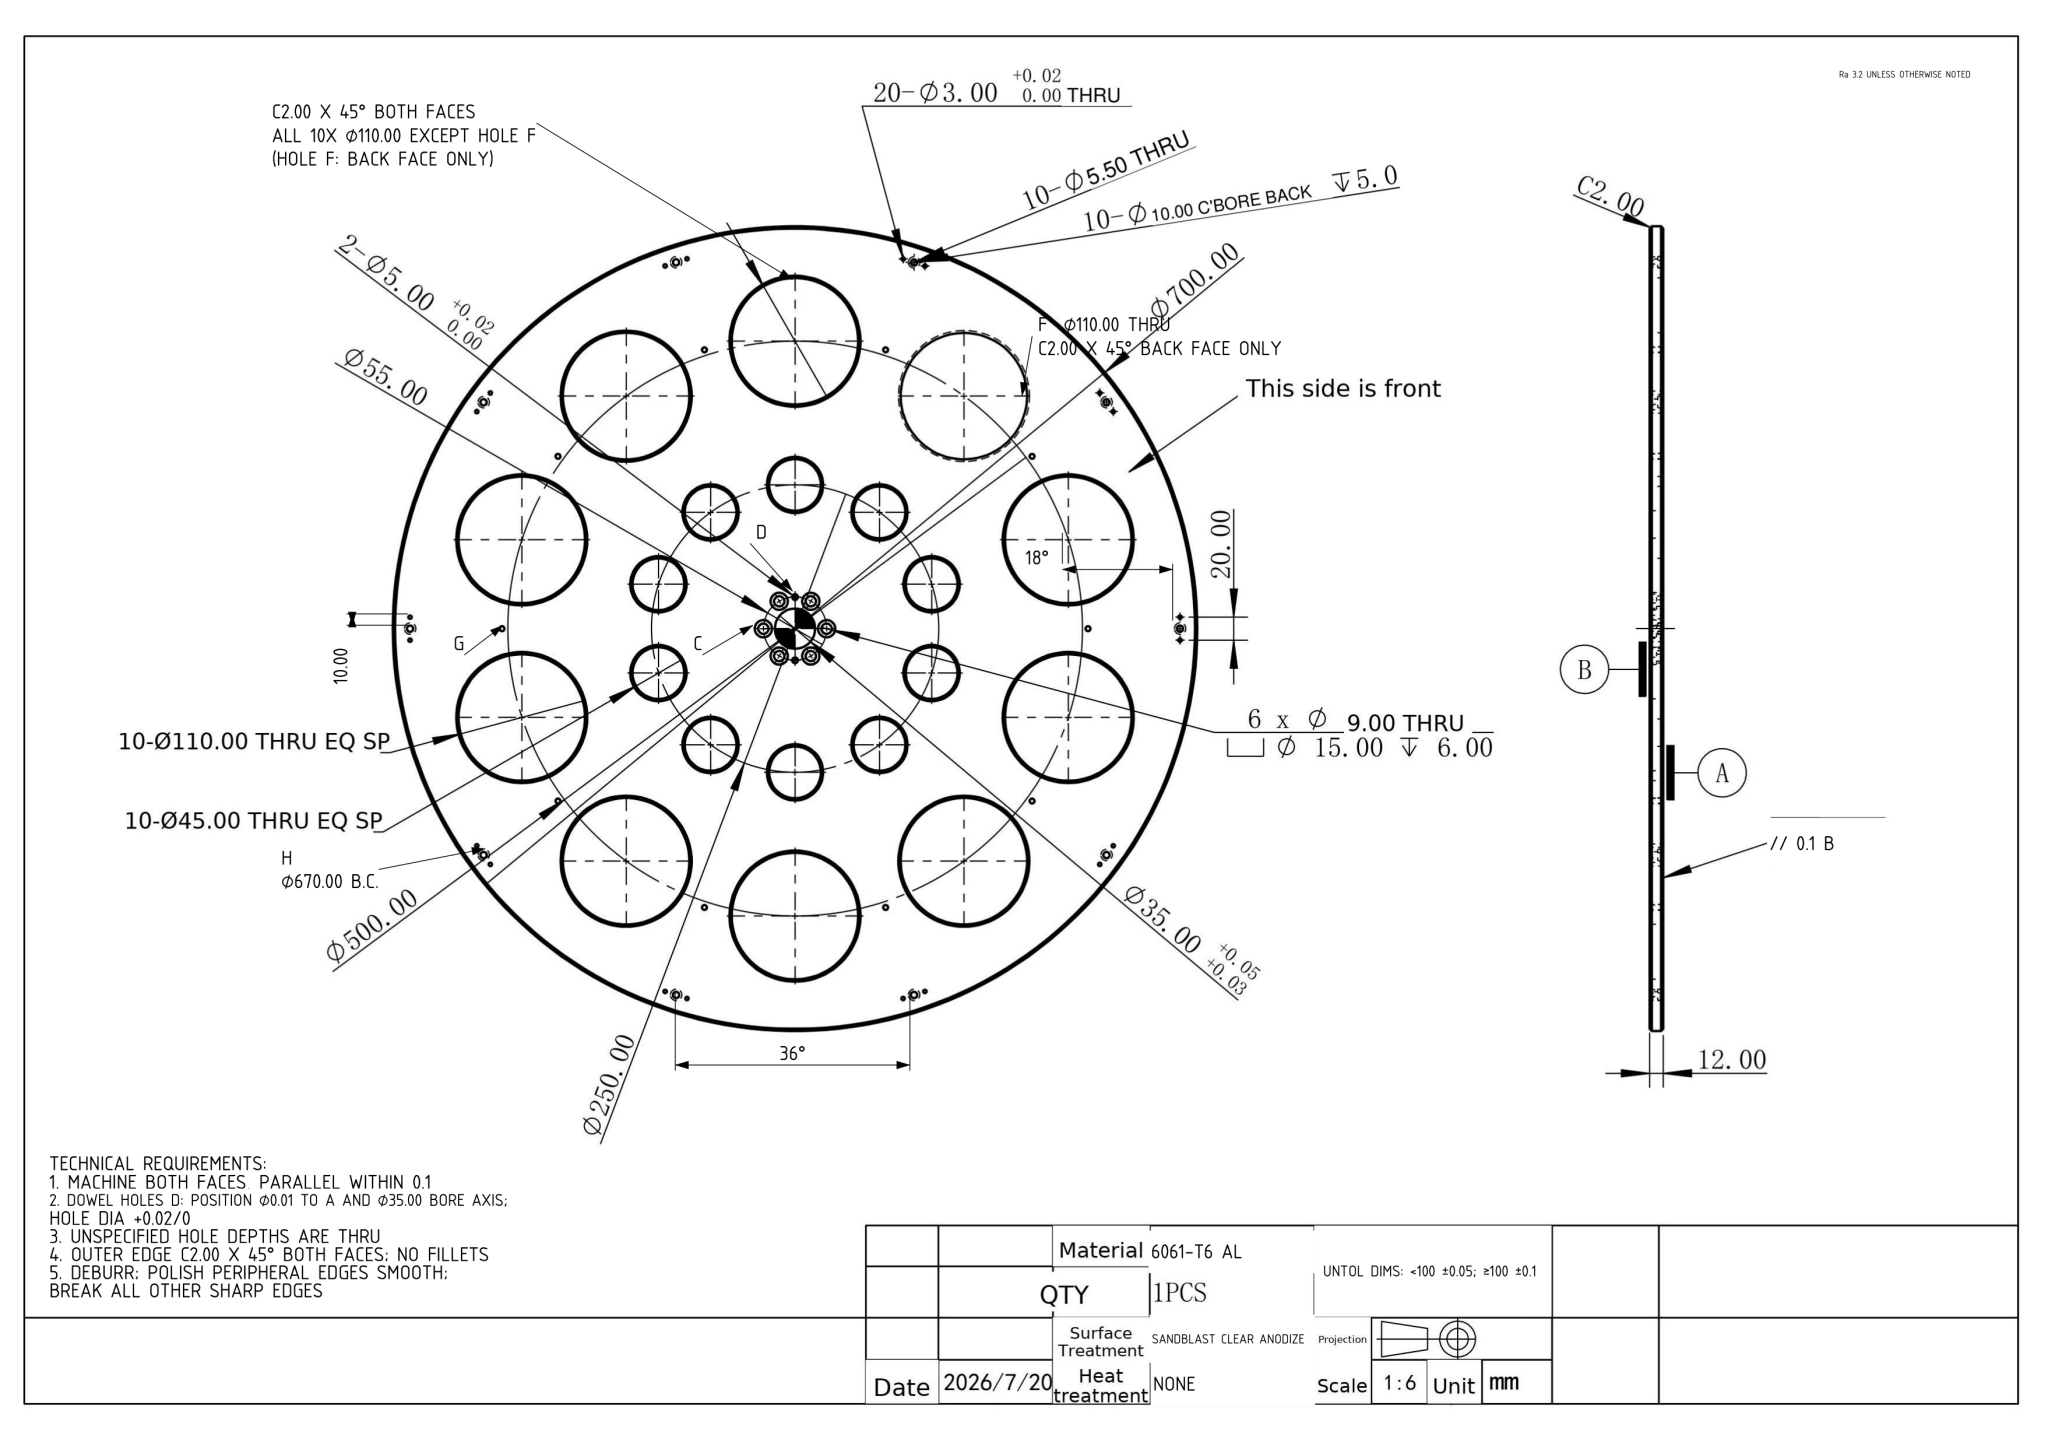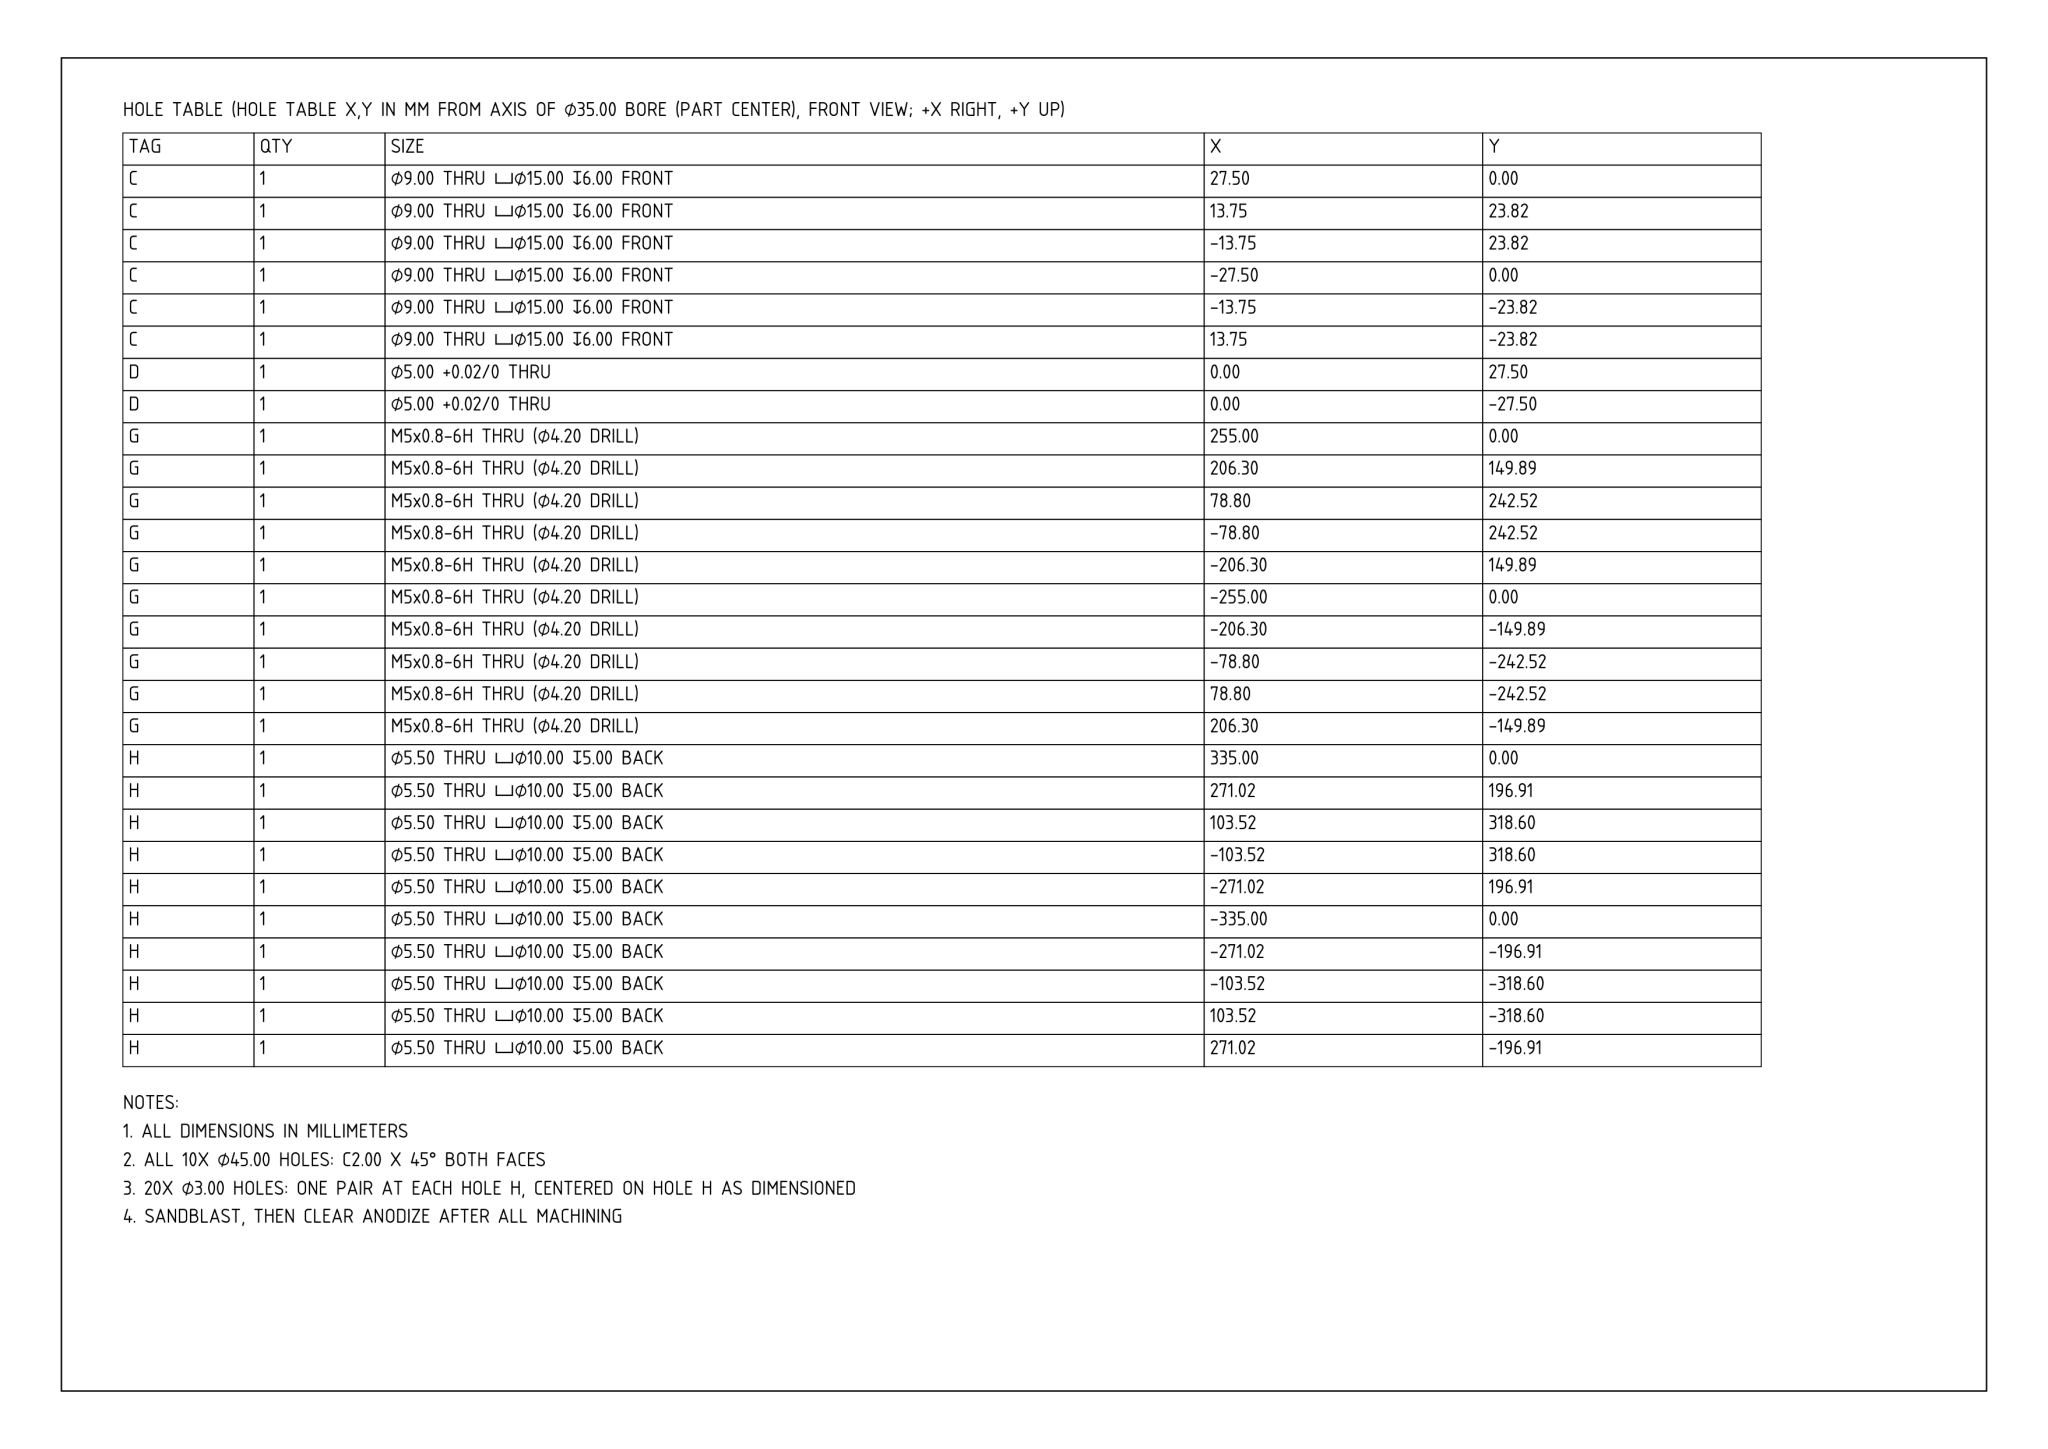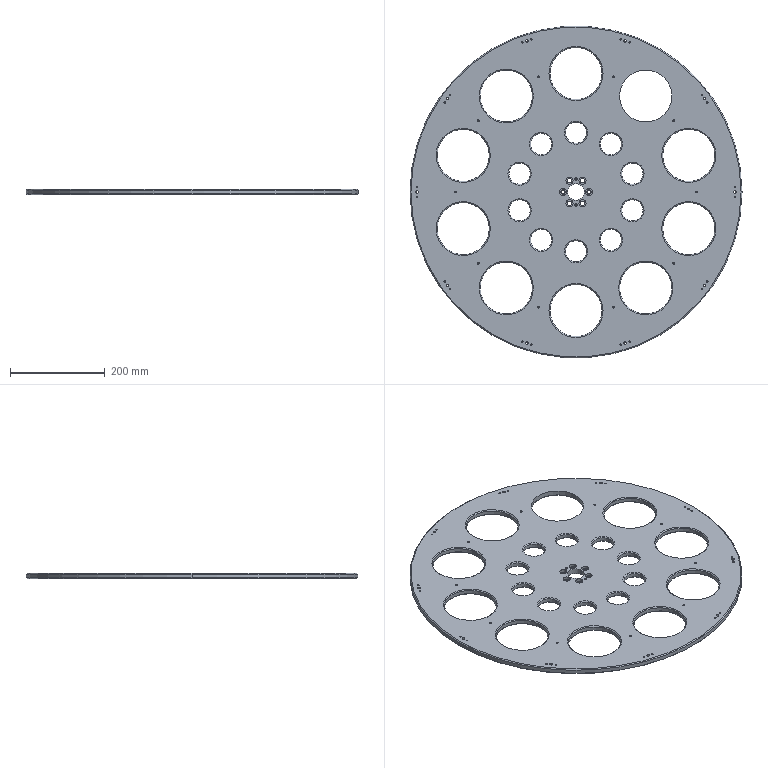Part | NX | mm | 1 solid | 272 faces | box 700 x 700 x 12 mm | volume 3229381 mm3 | cylinder 172 | cone 82 | plane 18 | commonest cylinder face diameters 3 x40 4.2 x20 10 x20 45 x20 110 x20 5.5 x20 15 x12 9 x12